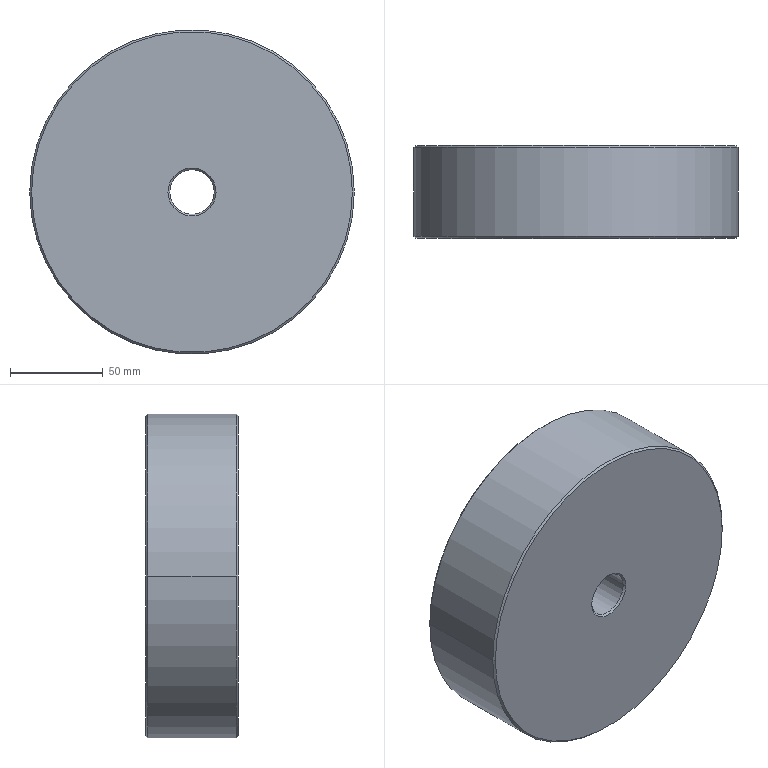Component | SolidWorks | LargePulley-1 | 1 solid | 14 faces | box 175 x 50 x 175 mm | volume 1179396 mm3 | cone 8 | cylinder 4 | plane 2 | commonest cylinder face diameters 24 x2 175 x2 | material 45
build123d program:
from build123d import *

# Parameters (mm, degrees)
SKETCH1_R           = 87.5
SKETCH1_R_2         = 12
BOSS_EXTRUDE1_DEPTH = 50
CHAMFER1_SIZE       = 1


with BuildPart() as part:
    # Sketch1 → Boss-Extrude1 (new body)
    with BuildSketch(Plane.XY):
        Circle(SKETCH1_R)
        Circle(SKETCH1_R_2, mode=Mode.SUBTRACT)
    extrude(amount=BOSS_EXTRUDE1_DEPTH)

    # Chamfer1
    chamfer1_edges = [part.edges().sort_by_distance(p)[0] for p in [
        (-87.5, 0, 0),
        (-87.5, 0, 50),
        (-12, 0, 0),
        (-12, 0, 50),
    ]]
    chamfer(chamfer1_edges, length=CHAMFER1_SIZE)


solid = part.part

# Placed as in the assembly
solid = solid.moved(Location((-371.359, -342.185, 1412), (90, 0, 0)))
STEP:
#1=CARTESIAN_POINT('',(-11.215,-15.44,55.591));
#2=VERTEX_POINT('',#1);
#3=CARTESIAN_POINT('',(-18.026,-15.44,55.591));
#4=VERTEX_POINT('',#3);
#5=CARTESIAN_POINT('',(-14.62,-15.44,55.591));
#6=DIRECTION('',(-0.,-1.,0.));
#7=DIRECTION('',(1.,0.,0.));
#8=AXIS2_PLACEMENT_3D('',#5,#6,#7);
#9=CIRCLE('',#8,3.406);
#10=EDGE_CURVE('',#2,#4,#9,.T.);
#11=ORIENTED_EDGE('',*,*,#10,.F.);
#12=CARTESIAN_POINT('',(-11.176,-15.401,55.591));
#13=VERTEX_POINT('',#12);
#14=CARTESIAN_POINT('',(-11.215,-15.44,55.591));
#15=DIRECTION('',(0.7071,0.7071,0.));
#16=VECTOR('',#15,39.37);
#17=LINE('',#14,#16);
#18=EDGE_CURVE('',#2,#13,#17,.T.);
#19=ORIENTED_EDGE('',*,*,#18,.T.);
#20=CARTESIAN_POINT('',(-18.065,-15.401,55.591));
#21=VERTEX_POINT('',#20);
#22=CARTESIAN_POINT('',(-14.62,-15.401,55.591));
#23=DIRECTION('',(0.,1.,0.));
#24=DIRECTION('',(1.,0.,0.));
#25=AXIS2_PLACEMENT_3D('',#22,#23,#24);
#26=CIRCLE('',#25,3.445);
#27=EDGE_CURVE('',#21,#13,#26,.T.);
#28=ORIENTED_EDGE('',*,*,#27,.F.);
#29=CARTESIAN_POINT('',(-18.026,-15.44,55.591));
#30=DIRECTION('',(-0.7071,0.7071,-0.));
#31=VECTOR('',#30,39.37);
#32=LINE('',#29,#31);
#33=EDGE_CURVE('',#4,#21,#32,.T.);
#34=ORIENTED_EDGE('',*,*,#33,.F.);
#35=EDGE_LOOP('',(#11,#19,#28,#34));
#36=FACE_OUTER_BOUND('',#35,.T.);
#37=CARTESIAN_POINT('',(-14.62,-15.44,55.591));
#38=DIRECTION('',(0.,1.,0.));
#39=DIRECTION('',(-1.,0.,0.));
#40=AXIS2_PLACEMENT_3D('',#37,#38,#39);
#41=CONICAL_SURFACE('',#40,3.406,0.7854);
#42=ADVANCED_FACE('',(#36),#41,.T.);
#43=CARTESIAN_POINT('',(-18.026,-13.472,55.591));
#44=VERTEX_POINT('',#43);
#45=CARTESIAN_POINT('',(-11.215,-13.472,55.591));
#46=VERTEX_POINT('',#45);
#47=CARTESIAN_POINT('',(-14.62,-13.472,55.591));
#48=DIRECTION('',(0.,1.,0.));
#49=DIRECTION('',(1.,0.,0.));
#50=AXIS2_PLACEMENT_3D('',#47,#48,#49);
#51=CIRCLE('',#50,3.406);
#52=EDGE_CURVE('',#44,#46,#51,.T.);
#53=ORIENTED_EDGE('',*,*,#52,.F.);
#54=CARTESIAN_POINT('',(-18.065,-13.511,55.591));
#55=VERTEX_POINT('',#54);
#56=CARTESIAN_POINT('',(-18.065,-13.511,55.591));
#57=DIRECTION('',(-0.7071,-0.7071,0.));
#58=VECTOR('',#57,39.37);
#59=LINE('',#56,#58);
#60=EDGE_CURVE('',#44,#55,#59,.T.);
#61=ORIENTED_EDGE('',*,*,#60,.T.);
#62=CARTESIAN_POINT('',(-11.176,-13.511,55.591));
#63=VERTEX_POINT('',#62);
#64=CARTESIAN_POINT('',(-14.62,-13.511,55.591));
#65=DIRECTION('',(-0.,-1.,0.));
#66=DIRECTION('',(1.,0.,0.));
#67=AXIS2_PLACEMENT_3D('',#64,#65,#66);
#68=CIRCLE('',#67,3.445);
#69=EDGE_CURVE('',#63,#55,#68,.T.);
#70=ORIENTED_EDGE('',*,*,#69,.F.);
#71=CARTESIAN_POINT('',(-11.176,-13.511,55.591));
#72=DIRECTION('',(0.7071,-0.7071,0.));
#73=VECTOR('',#72,39.37);
#74=LINE('',#71,#73);
#75=EDGE_CURVE('',#46,#63,#74,.T.);
#76=ORIENTED_EDGE('',*,*,#75,.F.);
#77=EDGE_LOOP('',(#53,#61,#70,#76));
#78=FACE_OUTER_BOUND('',#77,.T.);
#79=CARTESIAN_POINT('',(-14.62,-13.511,55.591));
#80=DIRECTION('',(-0.,-1.,0.));
#81=DIRECTION('',(1.,0.,0.));
#82=AXIS2_PLACEMENT_3D('',#79,#80,#81);
#83=CONICAL_SURFACE('',#82,3.445,0.7854);
#84=ADVANCED_FACE('',(#78),#83,.T.);
#85=CARTESIAN_POINT('',(-15.093,-15.401,55.591));
#86=VERTEX_POINT('',#85);
#87=CARTESIAN_POINT('',(-14.148,-15.401,55.591));
#88=VERTEX_POINT('',#87);
#89=CARTESIAN_POINT('',(-14.62,-15.401,55.591));
#90=DIRECTION('',(-0.,-1.,0.));
#91=DIRECTION('',(1.,0.,0.));
#92=AXIS2_PLACEMENT_3D('',#89,#90,#91);
#93=CIRCLE('',#92,0.4724);
#94=EDGE_CURVE('',#86,#88,#93,.T.);
#95=ORIENTED_EDGE('',*,*,#94,.F.);
#96=CARTESIAN_POINT('',(-15.132,-15.44,55.591));
#97=VERTEX_POINT('',#96);
#98=CARTESIAN_POINT('',(-15.093,-15.401,55.591));
#99=DIRECTION('',(-0.7071,-0.7071,0.));
#100=VECTOR('',#99,39.37);
#101=LINE('',#98,#100);
#102=EDGE_CURVE('',#86,#97,#101,.T.);
#103=ORIENTED_EDGE('',*,*,#102,.T.);
#104=CARTESIAN_POINT('',(-14.109,-15.44,55.591));
#105=VERTEX_POINT('',#104);
#106=CARTESIAN_POINT('',(-14.62,-15.44,55.591));
#107=DIRECTION('',(0.,1.,0.));
#108=DIRECTION('',(1.,0.,0.));
#109=AXIS2_PLACEMENT_3D('',#106,#107,#108);
#110=CIRCLE('',#109,0.5118);
#111=EDGE_CURVE('',#105,#97,#110,.T.);
#112=ORIENTED_EDGE('',*,*,#111,.F.);
#113=CARTESIAN_POINT('',(-14.148,-15.401,55.591));
#114=DIRECTION('',(0.7071,-0.7071,0.));
#115=VECTOR('',#114,39.37);
#116=LINE('',#113,#115);
#117=EDGE_CURVE('',#88,#105,#116,.T.);
#118=ORIENTED_EDGE('',*,*,#117,.F.);
#119=EDGE_LOOP('',(#95,#103,#112,#118));
#120=FACE_OUTER_BOUND('',#119,.T.);
#121=CARTESIAN_POINT('',(-14.62,-15.401,55.591));
#122=DIRECTION('',(-0.,-1.,0.));
#123=DIRECTION('',(1.,0.,0.));
#124=AXIS2_PLACEMENT_3D('',#121,#122,#123);
#125=CONICAL_SURFACE('',#124,0.4724,0.7854);
#126=ADVANCED_FACE('',(#120),#125,.F.);
#127=CARTESIAN_POINT('',(-14.148,-13.511,55.591));
#128=VERTEX_POINT('',#127);
#129=CARTESIAN_POINT('',(-15.093,-13.511,55.591));
#130=VERTEX_POINT('',#129);
#131=CARTESIAN_POINT('',(-14.62,-13.511,55.591));
#132=DIRECTION('',(0.,1.,0.));
#133=DIRECTION('',(1.,0.,0.));
#134=AXIS2_PLACEMENT_3D('',#131,#132,#133);
#135=CIRCLE('',#134,0.4724);
#136=EDGE_CURVE('',#128,#130,#135,.T.);
#137=ORIENTED_EDGE('',*,*,#136,.F.);
#138=CARTESIAN_POINT('',(-14.109,-13.472,55.591));
#139=VERTEX_POINT('',#138);
#140=CARTESIAN_POINT('',(-14.109,-13.472,55.591));
#141=DIRECTION('',(0.7071,0.7071,0.));
#142=VECTOR('',#141,39.37);
#143=LINE('',#140,#142);
#144=EDGE_CURVE('',#128,#139,#143,.T.);
#145=ORIENTED_EDGE('',*,*,#144,.T.);
#146=CARTESIAN_POINT('',(-15.132,-13.472,55.591));
#147=VERTEX_POINT('',#146);
#148=CARTESIAN_POINT('',(-14.62,-13.472,55.591));
#149=DIRECTION('',(-0.,-1.,0.));
#150=DIRECTION('',(1.,0.,0.));
#151=AXIS2_PLACEMENT_3D('',#148,#149,#150);
#152=CIRCLE('',#151,0.5118);
#153=EDGE_CURVE('',#147,#139,#152,.T.);
#154=ORIENTED_EDGE('',*,*,#153,.F.);
#155=CARTESIAN_POINT('',(-15.132,-13.472,55.591));
#156=DIRECTION('',(-0.7071,0.7071,-0.));
#157=VECTOR('',#156,39.37);
#158=LINE('',#155,#157);
#159=EDGE_CURVE('',#130,#147,#158,.T.);
#160=ORIENTED_EDGE('',*,*,#159,.F.);
#161=EDGE_LOOP('',(#137,#145,#154,#160));
#162=FACE_OUTER_BOUND('',#161,.T.);
#163=CARTESIAN_POINT('',(-14.62,-13.472,55.591));
#164=DIRECTION('',(0.,1.,0.));
#165=DIRECTION('',(-1.,0.,0.));
#166=AXIS2_PLACEMENT_3D('',#163,#164,#165);
#167=CONICAL_SURFACE('',#166,0.5118,0.7854);
#168=ADVANCED_FACE('',(#162),#167,.F.);
#169=ORIENTED_EDGE('',*,*,#94,.T.);
#170=CARTESIAN_POINT('',(-14.148,-15.44,55.591));
#171=DIRECTION('',(0.,1.,0.));
#172=VECTOR('',#171,39.37);
#173=LINE('',#170,#172);
#174=EDGE_CURVE('',#88,#128,#173,.T.);
#175=ORIENTED_EDGE('',*,*,#174,.T.);
#176=ORIENTED_EDGE('',*,*,#136,.T.);
#177=CARTESIAN_POINT('',(-15.093,-15.44,55.591));
#178=DIRECTION('',(0.,1.,0.));
#179=VECTOR('',#178,39.37);
#180=LINE('',#177,#179);
#181=EDGE_CURVE('',#86,#130,#180,.T.);
#182=ORIENTED_EDGE('',*,*,#181,.F.);
#183=EDGE_LOOP('',(#169,#175,#176,#182));
#184=FACE_OUTER_BOUND('',#183,.T.);
#185=CARTESIAN_POINT('',(-14.62,-15.44,55.591));
#186=DIRECTION('',(0.,1.,0.));
#187=DIRECTION('',(-1.,0.,0.));
#188=AXIS2_PLACEMENT_3D('',#185,#186,#187);
#189=CYLINDRICAL_SURFACE('',#188,0.4724);
#190=ADVANCED_FACE('',(#184),#189,.F.);
#191=ORIENTED_EDGE('',*,*,#27,.T.);
#192=CARTESIAN_POINT('',(-11.176,-15.44,55.591));
#193=DIRECTION('',(0.,1.,0.));
#194=VECTOR('',#193,39.37);
#195=LINE('',#192,#194);
#196=EDGE_CURVE('',#13,#63,#195,.T.);
#197=ORIENTED_EDGE('',*,*,#196,.T.);
#198=ORIENTED_EDGE('',*,*,#69,.T.);
#199=CARTESIAN_POINT('',(-18.065,-15.44,55.591));
#200=DIRECTION('',(0.,1.,0.));
#201=VECTOR('',#200,39.37);
#202=LINE('',#199,#201);
#203=EDGE_CURVE('',#21,#55,#202,.T.);
#204=ORIENTED_EDGE('',*,*,#203,.F.);
#205=EDGE_LOOP('',(#191,#197,#198,#204));
#206=FACE_OUTER_BOUND('',#205,.T.);
#207=CARTESIAN_POINT('',(-14.62,-15.44,55.591));
#208=DIRECTION('',(0.,1.,0.));
#209=DIRECTION('',(-1.,0.,0.));
#210=AXIS2_PLACEMENT_3D('',#207,#208,#209);
#211=CYLINDRICAL_SURFACE('',#210,3.445);
#212=ADVANCED_FACE('',(#206),#211,.T.);
#213=ORIENTED_EDGE('',*,*,#111,.T.);
#214=CARTESIAN_POINT('',(-14.62,-15.44,55.591));
#215=DIRECTION('',(0.,1.,0.));
#216=DIRECTION('',(1.,0.,0.));
#217=AXIS2_PLACEMENT_3D('',#214,#215,#216);
#218=CIRCLE('',#217,0.5118);
#219=EDGE_CURVE('',#97,#105,#218,.T.);
#220=ORIENTED_EDGE('',*,*,#219,.T.);
#221=EDGE_LOOP('',(#213,#220));
#222=FACE_BOUND('',#221,.T.);
#223=CARTESIAN_POINT('',(-14.62,-15.44,55.591));
#224=DIRECTION('',(-0.,-1.,0.));
#225=DIRECTION('',(1.,0.,0.));
#226=AXIS2_PLACEMENT_3D('',#223,#224,#225);
#227=CIRCLE('',#226,3.406);
#228=EDGE_CURVE('',#4,#2,#227,.T.);
#229=ORIENTED_EDGE('',*,*,#228,.T.);
#230=ORIENTED_EDGE('',*,*,#10,.T.);
#231=EDGE_LOOP('',(#229,#230));
#232=FACE_OUTER_BOUND('',#231,.T.);
#233=CARTESIAN_POINT('',(-14.62,-15.44,55.591));
#234=DIRECTION('',(-0.,-1.,0.));
#235=DIRECTION('',(1.,-0.,0.));
#236=AXIS2_PLACEMENT_3D('',#233,#234,#235);
#237=PLANE('',#236);
#238=ADVANCED_FACE('',(#222,#232),#237,.T.);
#239=ORIENTED_EDGE('',*,*,#153,.T.);
#240=CARTESIAN_POINT('',(-14.62,-13.472,55.591));
#241=DIRECTION('',(-0.,-1.,0.));
#242=DIRECTION('',(1.,0.,0.));
#243=AXIS2_PLACEMENT_3D('',#240,#241,#242);
#244=CIRCLE('',#243,0.5118);
#245=EDGE_CURVE('',#139,#147,#244,.T.);
#246=ORIENTED_EDGE('',*,*,#245,.T.);
#247=EDGE_LOOP('',(#239,#246));
#248=FACE_BOUND('',#247,.T.);
#249=CARTESIAN_POINT('',(-14.62,-13.472,55.591));
#250=DIRECTION('',(0.,1.,0.));
#251=DIRECTION('',(1.,0.,0.));
#252=AXIS2_PLACEMENT_3D('',#249,#250,#251);
#253=CIRCLE('',#252,3.406);
#254=EDGE_CURVE('',#46,#44,#253,.T.);
#255=ORIENTED_EDGE('',*,*,#254,.T.);
#256=ORIENTED_EDGE('',*,*,#52,.T.);
#257=EDGE_LOOP('',(#255,#256));
#258=FACE_OUTER_BOUND('',#257,.T.);
#259=CARTESIAN_POINT('',(-14.62,-13.472,55.591));
#260=DIRECTION('',(-0.,-1.,0.));
#261=DIRECTION('',(1.,-0.,0.));
#262=AXIS2_PLACEMENT_3D('',#259,#260,#261);
#263=PLANE('',#262);
#264=ADVANCED_FACE('',(#248,#258),#263,.F.);
#265=ORIENTED_EDGE('',*,*,#196,.F.);
#266=CARTESIAN_POINT('',(-14.62,-15.401,55.591));
#267=DIRECTION('',(0.,1.,0.));
#268=DIRECTION('',(1.,0.,0.));
#269=AXIS2_PLACEMENT_3D('',#266,#267,#268);
#270=CIRCLE('',#269,3.445);
#271=EDGE_CURVE('',#13,#21,#270,.T.);
#272=ORIENTED_EDGE('',*,*,#271,.T.);
#273=ORIENTED_EDGE('',*,*,#203,.T.);
#274=CARTESIAN_POINT('',(-14.62,-13.511,55.591));
#275=DIRECTION('',(-0.,-1.,0.));
#276=DIRECTION('',(1.,0.,0.));
#277=AXIS2_PLACEMENT_3D('',#274,#275,#276);
#278=CIRCLE('',#277,3.445);
#279=EDGE_CURVE('',#55,#63,#278,.T.);
#280=ORIENTED_EDGE('',*,*,#279,.T.);
#281=EDGE_LOOP('',(#265,#272,#273,#280));
#282=FACE_OUTER_BOUND('',#281,.T.);
#283=CARTESIAN_POINT('',(-14.62,-15.44,55.591));
#284=DIRECTION('',(0.,1.,0.));
#285=DIRECTION('',(-1.,0.,0.));
#286=AXIS2_PLACEMENT_3D('',#283,#284,#285);
#287=CYLINDRICAL_SURFACE('',#286,3.445);
#288=ADVANCED_FACE('',(#282),#287,.T.);
#289=ORIENTED_EDGE('',*,*,#174,.F.);
#290=CARTESIAN_POINT('',(-14.62,-15.401,55.591));
#291=DIRECTION('',(-0.,-1.,0.));
#292=DIRECTION('',(1.,0.,0.));
#293=AXIS2_PLACEMENT_3D('',#290,#291,#292);
#294=CIRCLE('',#293,0.4724);
#295=EDGE_CURVE('',#88,#86,#294,.T.);
#296=ORIENTED_EDGE('',*,*,#295,.T.);
#297=ORIENTED_EDGE('',*,*,#181,.T.);
#298=CARTESIAN_POINT('',(-14.62,-13.511,55.591));
#299=DIRECTION('',(0.,1.,0.));
#300=DIRECTION('',(1.,0.,0.));
#301=AXIS2_PLACEMENT_3D('',#298,#299,#300);
#302=CIRCLE('',#301,0.4724);
#303=EDGE_CURVE('',#130,#128,#302,.T.);
#304=ORIENTED_EDGE('',*,*,#303,.T.);
#305=EDGE_LOOP('',(#289,#296,#297,#304));
#306=FACE_OUTER_BOUND('',#305,.T.);
#307=CARTESIAN_POINT('',(-14.62,-15.44,55.591));
#308=DIRECTION('',(0.,1.,0.));
#309=DIRECTION('',(-1.,0.,0.));
#310=AXIS2_PLACEMENT_3D('',#307,#308,#309);
#311=CYLINDRICAL_SURFACE('',#310,0.4724);
#312=ADVANCED_FACE('',(#306),#311,.F.);
#313=ORIENTED_EDGE('',*,*,#144,.F.);
#314=ORIENTED_EDGE('',*,*,#303,.F.);
#315=ORIENTED_EDGE('',*,*,#159,.T.);
#316=ORIENTED_EDGE('',*,*,#245,.F.);
#317=EDGE_LOOP('',(#313,#314,#315,#316));
#318=FACE_OUTER_BOUND('',#317,.T.);
#319=CARTESIAN_POINT('',(-14.62,-13.472,55.591));
#320=DIRECTION('',(0.,1.,0.));
#321=DIRECTION('',(-1.,0.,0.));
#322=AXIS2_PLACEMENT_3D('',#319,#320,#321);
#323=CONICAL_SURFACE('',#322,0.5118,0.7854);
#324=ADVANCED_FACE('',(#318),#323,.F.);
#325=ORIENTED_EDGE('',*,*,#102,.F.);
#326=ORIENTED_EDGE('',*,*,#295,.F.);
#327=ORIENTED_EDGE('',*,*,#117,.T.);
#328=ORIENTED_EDGE('',*,*,#219,.F.);
#329=EDGE_LOOP('',(#325,#326,#327,#328));
#330=FACE_OUTER_BOUND('',#329,.T.);
#331=CARTESIAN_POINT('',(-14.62,-15.401,55.591));
#332=DIRECTION('',(-0.,-1.,0.));
#333=DIRECTION('',(1.,0.,0.));
#334=AXIS2_PLACEMENT_3D('',#331,#332,#333);
#335=CONICAL_SURFACE('',#334,0.4724,0.7854);
#336=ADVANCED_FACE('',(#330),#335,.F.);
#337=ORIENTED_EDGE('',*,*,#60,.F.);
#338=ORIENTED_EDGE('',*,*,#254,.F.);
#339=ORIENTED_EDGE('',*,*,#75,.T.);
#340=ORIENTED_EDGE('',*,*,#279,.F.);
#341=EDGE_LOOP('',(#337,#338,#339,#340));
#342=FACE_OUTER_BOUND('',#341,.T.);
#343=CARTESIAN_POINT('',(-14.62,-13.511,55.591));
#344=DIRECTION('',(-0.,-1.,0.));
#345=DIRECTION('',(1.,0.,0.));
#346=AXIS2_PLACEMENT_3D('',#343,#344,#345);
#347=CONICAL_SURFACE('',#346,3.445,0.7854);
#348=ADVANCED_FACE('',(#342),#347,.T.);
#349=ORIENTED_EDGE('',*,*,#18,.F.);
#350=ORIENTED_EDGE('',*,*,#228,.F.);
#351=ORIENTED_EDGE('',*,*,#33,.T.);
#352=ORIENTED_EDGE('',*,*,#271,.F.);
#353=EDGE_LOOP('',(#349,#350,#351,#352));
#354=FACE_OUTER_BOUND('',#353,.T.);
#355=CARTESIAN_POINT('',(-14.62,-15.44,55.591));
#356=DIRECTION('',(0.,1.,0.));
#357=DIRECTION('',(-1.,0.,0.));
#358=AXIS2_PLACEMENT_3D('',#355,#356,#357);
#359=CONICAL_SURFACE('',#358,3.406,0.7854);
#360=ADVANCED_FACE('',(#354),#359,.T.);
#361=CLOSED_SHELL('',(#42,#84,#126,#168,#190,#212,#238,#264,#288,#312,#324,#336,#348,#360));
#362=MANIFOLD_SOLID_BREP('',#361);
#363=CARTESIAN_POINT('',(0.,0.,0.));
#364=DIRECTION('',(0.,0.,1.));
#365=DIRECTION('',(1.,0.,0.));
#366=AXIS2_PLACEMENT_3D('',#363,#364,#365);
#367=(LENGTH_UNIT()NAMED_UNIT(*)SI_UNIT($,.METRE.));
#368=LENGTH_MEASURE_WITH_UNIT(LENGTH_MEASURE(0.0254),#367);
#369=DIMENSIONAL_EXPONENTS(1.,0.,0.,0.,0.,0.,0.);
#370=(CONVERSION_BASED_UNIT('',#368)LENGTH_UNIT()NAMED_UNIT(#369));
#371=UNCERTAINTY_MEASURE_WITH_UNIT(LENGTH_MEASURE(0.00001),#370,'','');
#372=(NAMED_UNIT(*)PLANE_ANGLE_UNIT()SI_UNIT($,.RADIAN.));
#373=(NAMED_UNIT(*)SI_UNIT($,.STERADIAN.)SOLID_ANGLE_UNIT());
#374=(GEOMETRIC_REPRESENTATION_CONTEXT(3)GLOBAL_UNCERTAINTY_ASSIGNED_CONTEXT((#371))GLOBAL_UNIT_ASSIGNED_CONTEXT((#370,#372,#373))REPRESENTATION_CONTEXT('',''));
#375=ADVANCED_BREP_SHAPE_REPRESENTATION('',(#362,#366),#374);
#376=COLOUR_RGB('',0.7922,0.8196,0.9333);
#377=FILL_AREA_STYLE_COLOUR('',#376);
#378=FILL_AREA_STYLE('',(#377));
#379=SURFACE_STYLE_FILL_AREA(#378);
#380=SURFACE_SIDE_STYLE('',(#379));
#381=SURFACE_STYLE_USAGE(.BOTH.,#380);
#382=PRESENTATION_STYLE_ASSIGNMENT((#381));
#383=STYLED_ITEM('',(#382),#362);
#384=PRESENTATION_LAYER_ASSIGNMENT('','',(#383));
#385=(LENGTH_UNIT()NAMED_UNIT(*)SI_UNIT($,.METRE.));
#386=LENGTH_MEASURE_WITH_UNIT(LENGTH_MEASURE(0.0254),#385);
#387=DIMENSIONAL_EXPONENTS(1.,0.,0.,0.,0.,0.,0.);
#388=(CONVERSION_BASED_UNIT('',#386)LENGTH_UNIT()NAMED_UNIT(#387));
#389=UNCERTAINTY_MEASURE_WITH_UNIT(LENGTH_MEASURE(0.00001),#388,'','');
#390=(NAMED_UNIT(*)PLANE_ANGLE_UNIT()SI_UNIT($,.RADIAN.));
#391=(NAMED_UNIT(*)SI_UNIT($,.STERADIAN.)SOLID_ANGLE_UNIT());
#392=(GEOMETRIC_REPRESENTATION_CONTEXT(3)GLOBAL_UNCERTAINTY_ASSIGNED_CONTEXT((#389))GLOBAL_UNIT_ASSIGNED_CONTEXT((#388,#390,#391))REPRESENTATION_CONTEXT('',''));
#393=MECHANICAL_DESIGN_GEOMETRIC_PRESENTATION_REPRESENTATION('',(#383),#392);